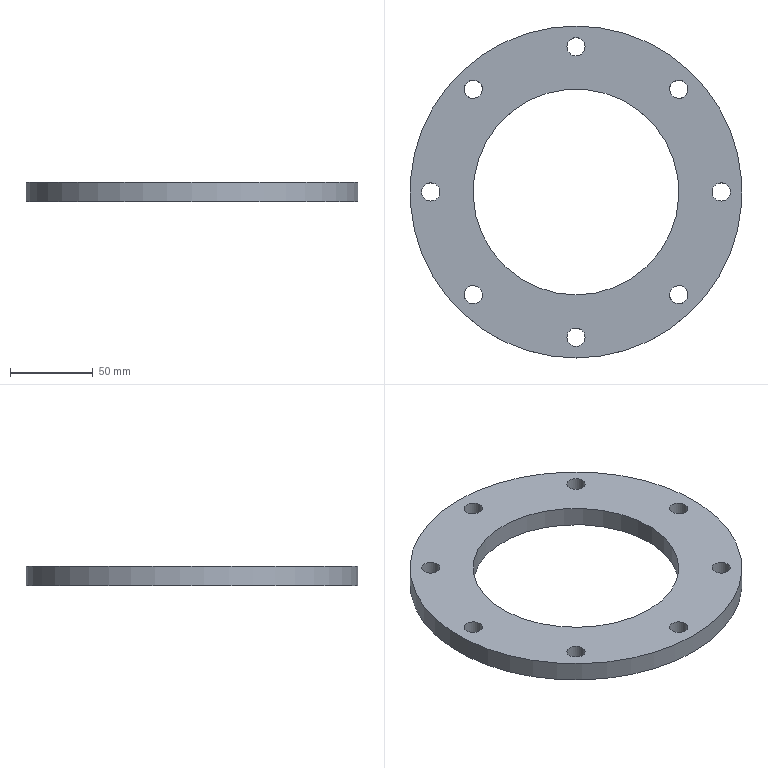Component | NX | CH3404_8_2-2 | 1 solid | 12 faces | volume 222953 mm3 | cylinder 10 | plane 2 | commonest cylinder face diameters 11 x8 200 x1 124 x1